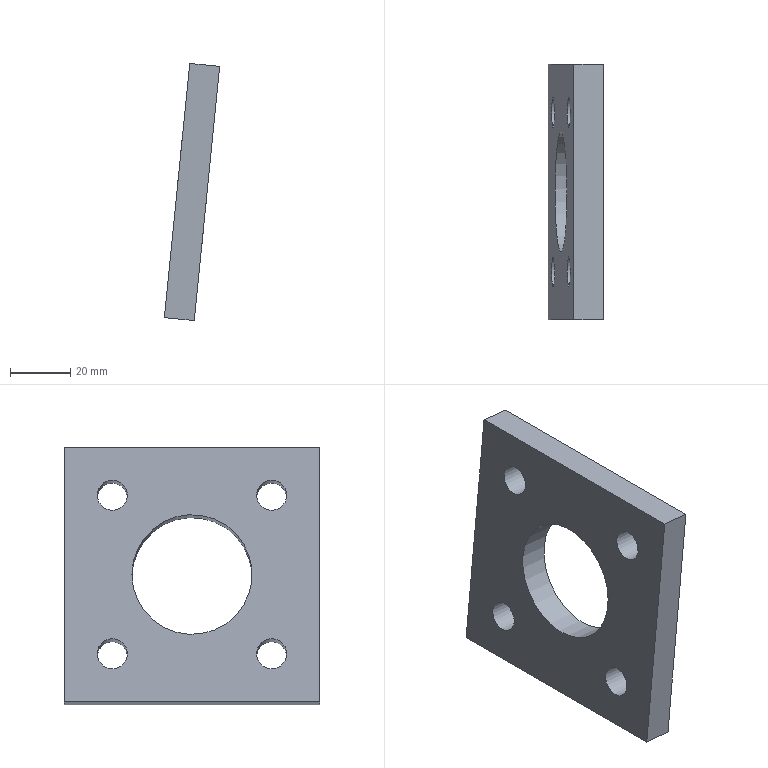Component | NX | UP_FRAME_BLOCK_2 | 1 solid | 11 faces | box 18.39 x 85 x 85.57 mm | volume 56542 mm3 | plane 6 | cylinder 5 | commonest cylinder face diameters 10 x4 40 x1
STEP:
#1=CARTESIAN_POINT('',(0.,0.,0.));
#2=DIRECTION('',(0.,0.,1.));
#3=DIRECTION('',(1.,0.,0.));
#4=AXIS2_PLACEMENT_3D('',#1,#2,#3);
#5=CARTESIAN_POINT('',(1555.629,25.,356.975));
#6=VERTEX_POINT('',#5);
#7=CARTESIAN_POINT('',(1564.071,25.,441.554));
#8=VERTEX_POINT('',#7);
#9=CARTESIAN_POINT('',(1555.629,25.,356.975));
#10=DIRECTION('',(0.09932,-0.,0.9951));
#11=VECTOR('',#10,1.);
#12=LINE('',#9,#11);
#13=CARTESIAN_POINT('',(1565.579,25.,355.981));
#14=DIRECTION('',(-0.,-1.,-0.));
#15=DIRECTION('',(-0.09932,0.,-0.9951));
#16=AXIS2_PLACEMENT_3D('',#13,#14,#15);
#17=PLANE('',#16);
#18=CARTESIAN_POINT('',(-0.,-10.));
#19=DIRECTION('',(-1.,0.));
#20=VECTOR('',#19,1.);
#21=LINE('',#18,#20);
#22=(GEOMETRIC_REPRESENTATION_CONTEXT(2)PARAMETRIC_REPRESENTATION_CONTEXT()REPRESENTATION_CONTEXT('',''));
#23=DEFINITIONAL_REPRESENTATION('',(#21),#22);
#24=PCURVE('',#17,#23);
#25=CARTESIAN_POINT('',(1562.484,94.017,425.65));
#26=DIRECTION('',(-0.9951,0.,0.09932));
#27=DIRECTION('',(0.09932,0.,0.9951));
#28=AXIS2_PLACEMENT_3D('',#25,#26,#27);
#29=PLANE('',#28);
#30=CARTESIAN_POINT('',(-69.017,-69.017));
#31=DIRECTION('',(1.,-0.));
#32=VECTOR('',#31,1.);
#33=LINE('',#30,#32);
#34=(GEOMETRIC_REPRESENTATION_CONTEXT(2)PARAMETRIC_REPRESENTATION_CONTEXT()REPRESENTATION_CONTEXT('',''));
#35=DEFINITIONAL_REPRESENTATION('',(#33),#34);
#36=PCURVE('',#29,#35);
#37=SURFACE_CURVE('',#12,(#24,#36),.PCURVE_S1.);
#38=EDGE_CURVE('',#6,#8,#37,.T.);
#39=ORIENTED_EDGE('',*,*,#38,.F.);
#40=CARTESIAN_POINT('',(1565.579,25.,355.981));
#41=VERTEX_POINT('',#40);
#42=CARTESIAN_POINT('',(1565.579,25.,355.981));
#43=DIRECTION('',(-0.9951,0.,0.09932));
#44=VECTOR('',#43,1.);
#45=LINE('',#42,#44);
#46=CARTESIAN_POINT('',(0.,0.));
#47=DIRECTION('',(0.,-1.));
#48=VECTOR('',#47,1.);
#49=LINE('',#46,#48);
#50=(GEOMETRIC_REPRESENTATION_CONTEXT(2)PARAMETRIC_REPRESENTATION_CONTEXT()REPRESENTATION_CONTEXT('',''));
#51=DEFINITIONAL_REPRESENTATION('',(#49),#50);
#52=PCURVE('',#17,#51);
#53=CARTESIAN_POINT('',(1565.579,110.,355.981));
#54=DIRECTION('',(-0.09932,0.,-0.9951));
#55=DIRECTION('',(-0.9951,0.,0.09932));
#56=AXIS2_PLACEMENT_3D('',#53,#54,#55);
#57=PLANE('',#56);
#58=CARTESIAN_POINT('',(0.,-85.));
#59=DIRECTION('',(1.,0.));
#60=VECTOR('',#59,1.);
#61=LINE('',#58,#60);
#62=(GEOMETRIC_REPRESENTATION_CONTEXT(2)PARAMETRIC_REPRESENTATION_CONTEXT()REPRESENTATION_CONTEXT('',''));
#63=DEFINITIONAL_REPRESENTATION('',(#61),#62);
#64=PCURVE('',#57,#63);
#65=SURFACE_CURVE('',#45,(#52,#64),.PCURVE_S1.);
#66=EDGE_CURVE('',#41,#6,#65,.T.);
#67=ORIENTED_EDGE('',*,*,#66,.F.);
#68=CARTESIAN_POINT('',(1574.022,25.,440.561));
#69=VERTEX_POINT('',#68);
#70=CARTESIAN_POINT('',(1565.579,25.,355.981));
#71=DIRECTION('',(0.09932,-0.,0.9951));
#72=VECTOR('',#71,1.);
#73=LINE('',#70,#72);
#74=CARTESIAN_POINT('',(0.,0.));
#75=DIRECTION('',(-1.,0.));
#76=VECTOR('',#75,1.);
#77=LINE('',#74,#76);
#78=(GEOMETRIC_REPRESENTATION_CONTEXT(2)PARAMETRIC_REPRESENTATION_CONTEXT()REPRESENTATION_CONTEXT('',''));
#79=DEFINITIONAL_REPRESENTATION('',(#77),#78);
#80=PCURVE('',#17,#79);
#81=CARTESIAN_POINT('',(1572.434,94.017,424.657));
#82=DIRECTION('',(-0.9951,0.,0.09932));
#83=DIRECTION('',(0.09932,0.,0.9951));
#84=AXIS2_PLACEMENT_3D('',#81,#82,#83);
#85=PLANE('',#84);
#86=CARTESIAN_POINT('',(-69.017,-69.017));
#87=DIRECTION('',(1.,-0.));
#88=VECTOR('',#87,1.);
#89=LINE('',#86,#88);
#90=(GEOMETRIC_REPRESENTATION_CONTEXT(2)PARAMETRIC_REPRESENTATION_CONTEXT()REPRESENTATION_CONTEXT('',''));
#91=DEFINITIONAL_REPRESENTATION('',(#89),#90);
#92=PCURVE('',#85,#91);
#93=SURFACE_CURVE('',#73,(#80,#92),.PCURVE_S1.);
#94=EDGE_CURVE('',#41,#69,#93,.T.);
#95=ORIENTED_EDGE('',*,*,#94,.T.);
#96=CARTESIAN_POINT('',(1574.022,25.,440.561));
#97=DIRECTION('',(-0.9951,0.,0.09932));
#98=VECTOR('',#97,1.);
#99=LINE('',#96,#98);
#100=CARTESIAN_POINT('',(-85.,0.));
#101=DIRECTION('',(0.,-1.));
#102=VECTOR('',#101,1.);
#103=LINE('',#100,#102);
#104=(GEOMETRIC_REPRESENTATION_CONTEXT(2)PARAMETRIC_REPRESENTATION_CONTEXT()REPRESENTATION_CONTEXT('',''));
#105=DEFINITIONAL_REPRESENTATION('',(#103),#104);
#106=PCURVE('',#17,#105);
#107=CARTESIAN_POINT('',(1574.022,25.,440.561));
#108=DIRECTION('',(0.09932,0.,0.9951));
#109=DIRECTION('',(0.9951,0.,-0.09932));
#110=AXIS2_PLACEMENT_3D('',#107,#108,#109);
#111=PLANE('',#110);
#112=CARTESIAN_POINT('',(0.,0.));
#113=DIRECTION('',(-1.,0.));
#114=VECTOR('',#113,1.);
#115=LINE('',#112,#114);
#116=(GEOMETRIC_REPRESENTATION_CONTEXT(2)PARAMETRIC_REPRESENTATION_CONTEXT()REPRESENTATION_CONTEXT('',''));
#117=DEFINITIONAL_REPRESENTATION('',(#115),#116);
#118=PCURVE('',#111,#117);
#119=SURFACE_CURVE('',#99,(#106,#118),.PCURVE_S1.);
#120=EDGE_CURVE('',#69,#8,#119,.T.);
#121=ORIENTED_EDGE('',*,*,#120,.T.);
#122=EDGE_LOOP('',(#39,#67,#95,#121));
#123=FACE_BOUND('',#122,.T.);
#124=ADVANCED_FACE('',(#123),#17,.T.);
#125=CARTESIAN_POINT('',(1564.071,110.,441.554));
#126=VERTEX_POINT('',#125);
#127=CARTESIAN_POINT('',(1564.071,25.,441.554));
#128=DIRECTION('',(0.,1.,0.));
#129=VECTOR('',#128,1.);
#130=LINE('',#127,#129);
#131=CARTESIAN_POINT('',(-10.,0.));
#132=DIRECTION('',(0.,1.));
#133=VECTOR('',#132,1.);
#134=LINE('',#131,#133);
#135=(GEOMETRIC_REPRESENTATION_CONTEXT(2)PARAMETRIC_REPRESENTATION_CONTEXT()REPRESENTATION_CONTEXT('',''));
#136=DEFINITIONAL_REPRESENTATION('',(#134),#135);
#137=PCURVE('',#111,#136);
#138=CARTESIAN_POINT('',(15.983,-69.017));
#139=DIRECTION('',(0.,1.));
#140=VECTOR('',#139,1.);
#141=LINE('',#138,#140);
#142=(GEOMETRIC_REPRESENTATION_CONTEXT(2)PARAMETRIC_REPRESENTATION_CONTEXT()REPRESENTATION_CONTEXT('',''));
#143=DEFINITIONAL_REPRESENTATION('',(#141),#142);
#144=PCURVE('',#29,#143);
#145=SURFACE_CURVE('',#130,(#137,#144),.PCURVE_S1.);
#146=EDGE_CURVE('',#8,#126,#145,.T.);
#147=ORIENTED_EDGE('',*,*,#146,.F.);
#148=ORIENTED_EDGE('',*,*,#120,.F.);
#149=CARTESIAN_POINT('',(1574.022,110.,440.561));
#150=VERTEX_POINT('',#149);
#151=CARTESIAN_POINT('',(1574.022,25.,440.561));
#152=DIRECTION('',(0.,1.,0.));
#153=VECTOR('',#152,1.);
#154=LINE('',#151,#153);
#155=CARTESIAN_POINT('',(0.,0.));
#156=DIRECTION('',(0.,1.));
#157=VECTOR('',#156,1.);
#158=LINE('',#155,#157);
#159=(GEOMETRIC_REPRESENTATION_CONTEXT(2)PARAMETRIC_REPRESENTATION_CONTEXT()REPRESENTATION_CONTEXT('',''));
#160=DEFINITIONAL_REPRESENTATION('',(#158),#159);
#161=PCURVE('',#111,#160);
#162=CARTESIAN_POINT('',(15.983,-69.017));
#163=DIRECTION('',(0.,1.));
#164=VECTOR('',#163,1.);
#165=LINE('',#162,#164);
#166=(GEOMETRIC_REPRESENTATION_CONTEXT(2)PARAMETRIC_REPRESENTATION_CONTEXT()REPRESENTATION_CONTEXT('',''));
#167=DEFINITIONAL_REPRESENTATION('',(#165),#166);
#168=PCURVE('',#85,#167);
#169=SURFACE_CURVE('',#154,(#161,#168),.PCURVE_S1.);
#170=EDGE_CURVE('',#69,#150,#169,.T.);
#171=ORIENTED_EDGE('',*,*,#170,.T.);
#172=CARTESIAN_POINT('',(1574.022,110.,440.561));
#173=DIRECTION('',(-0.9951,0.,0.09932));
#174=VECTOR('',#173,1.);
#175=LINE('',#172,#174);
#176=CARTESIAN_POINT('',(0.,85.));
#177=DIRECTION('',(-1.,0.));
#178=VECTOR('',#177,1.);
#179=LINE('',#176,#178);
#180=(GEOMETRIC_REPRESENTATION_CONTEXT(2)PARAMETRIC_REPRESENTATION_CONTEXT()REPRESENTATION_CONTEXT('',''));
#181=DEFINITIONAL_REPRESENTATION('',(#179),#180);
#182=PCURVE('',#111,#181);
#183=CARTESIAN_POINT('',(1574.022,110.,440.561));
#184=DIRECTION('',(0.,1.,0.));
#185=DIRECTION('',(0.09932,-0.,0.9951));
#186=AXIS2_PLACEMENT_3D('',#183,#184,#185);
#187=PLANE('',#186);
#188=CARTESIAN_POINT('',(0.,0.));
#189=DIRECTION('',(-0.,-1.));
#190=VECTOR('',#189,1.);
#191=LINE('',#188,#190);
#192=(GEOMETRIC_REPRESENTATION_CONTEXT(2)PARAMETRIC_REPRESENTATION_CONTEXT()REPRESENTATION_CONTEXT('',''));
#193=DEFINITIONAL_REPRESENTATION('',(#191),#192);
#194=PCURVE('',#187,#193);
#195=SURFACE_CURVE('',#175,(#182,#194),.PCURVE_S1.);
#196=EDGE_CURVE('',#150,#126,#195,.T.);
#197=ORIENTED_EDGE('',*,*,#196,.T.);
#198=EDGE_LOOP('',(#147,#148,#171,#197));
#199=FACE_BOUND('',#198,.T.);
#200=ADVANCED_FACE('',(#199),#111,.T.);
#201=CARTESIAN_POINT('',(1555.629,110.,356.975));
#202=VERTEX_POINT('',#201);
#203=CARTESIAN_POINT('',(1564.071,110.,441.554));
#204=DIRECTION('',(-0.09932,0.,-0.9951));
#205=VECTOR('',#204,1.);
#206=LINE('',#203,#205);
#207=CARTESIAN_POINT('',(0.,-10.));
#208=DIRECTION('',(-1.,0.));
#209=VECTOR('',#208,1.);
#210=LINE('',#207,#209);
#211=(GEOMETRIC_REPRESENTATION_CONTEXT(2)PARAMETRIC_REPRESENTATION_CONTEXT()REPRESENTATION_CONTEXT('',''));
#212=DEFINITIONAL_REPRESENTATION('',(#210),#211);
#213=PCURVE('',#187,#212);
#214=CARTESIAN_POINT('',(15.983,15.983));
#215=DIRECTION('',(-1.,0.));
#216=VECTOR('',#215,1.);
#217=LINE('',#214,#216);
#218=(GEOMETRIC_REPRESENTATION_CONTEXT(2)PARAMETRIC_REPRESENTATION_CONTEXT()REPRESENTATION_CONTEXT('',''));
#219=DEFINITIONAL_REPRESENTATION('',(#217),#218);
#220=PCURVE('',#29,#219);
#221=SURFACE_CURVE('',#206,(#213,#220),.PCURVE_S1.);
#222=EDGE_CURVE('',#126,#202,#221,.T.);
#223=ORIENTED_EDGE('',*,*,#222,.F.);
#224=ORIENTED_EDGE('',*,*,#196,.F.);
#225=CARTESIAN_POINT('',(1565.579,110.,355.981));
#226=VERTEX_POINT('',#225);
#227=CARTESIAN_POINT('',(1574.022,110.,440.561));
#228=DIRECTION('',(-0.09932,0.,-0.9951));
#229=VECTOR('',#228,1.);
#230=LINE('',#227,#229);
#231=CARTESIAN_POINT('',(0.,0.));
#232=DIRECTION('',(-1.,0.));
#233=VECTOR('',#232,1.);
#234=LINE('',#231,#233);
#235=(GEOMETRIC_REPRESENTATION_CONTEXT(2)PARAMETRIC_REPRESENTATION_CONTEXT()REPRESENTATION_CONTEXT('',''));
#236=DEFINITIONAL_REPRESENTATION('',(#234),#235);
#237=PCURVE('',#187,#236);
#238=CARTESIAN_POINT('',(15.983,15.983));
#239=DIRECTION('',(-1.,0.));
#240=VECTOR('',#239,1.);
#241=LINE('',#238,#240);
#242=(GEOMETRIC_REPRESENTATION_CONTEXT(2)PARAMETRIC_REPRESENTATION_CONTEXT()REPRESENTATION_CONTEXT('',''));
#243=DEFINITIONAL_REPRESENTATION('',(#241),#242);
#244=PCURVE('',#85,#243);
#245=SURFACE_CURVE('',#230,(#237,#244),.PCURVE_S1.);
#246=EDGE_CURVE('',#150,#226,#245,.T.);
#247=ORIENTED_EDGE('',*,*,#246,.T.);
#248=CARTESIAN_POINT('',(1565.579,110.,355.981));
#249=DIRECTION('',(-0.9951,0.,0.09932));
#250=VECTOR('',#249,1.);
#251=LINE('',#248,#250);
#252=CARTESIAN_POINT('',(-85.,-0.));
#253=DIRECTION('',(-0.,-1.));
#254=VECTOR('',#253,1.);
#255=LINE('',#252,#254);
#256=(GEOMETRIC_REPRESENTATION_CONTEXT(2)PARAMETRIC_REPRESENTATION_CONTEXT()REPRESENTATION_CONTEXT('',''));
#257=DEFINITIONAL_REPRESENTATION('',(#255),#256);
#258=PCURVE('',#187,#257);
#259=CARTESIAN_POINT('',(0.,0.));
#260=DIRECTION('',(1.,0.));
#261=VECTOR('',#260,1.);
#262=LINE('',#259,#261);
#263=(GEOMETRIC_REPRESENTATION_CONTEXT(2)PARAMETRIC_REPRESENTATION_CONTEXT()REPRESENTATION_CONTEXT('',''));
#264=DEFINITIONAL_REPRESENTATION('',(#262),#263);
#265=PCURVE('',#57,#264);
#266=SURFACE_CURVE('',#251,(#258,#265),.PCURVE_S1.);
#267=EDGE_CURVE('',#226,#202,#266,.T.);
#268=ORIENTED_EDGE('',*,*,#267,.T.);
#269=EDGE_LOOP('',(#223,#224,#247,#268));
#270=FACE_BOUND('',#269,.T.);
#271=ADVANCED_FACE('',(#270),#187,.T.);
#272=CARTESIAN_POINT('',(1572.434,45.983,424.657));
#273=VERTEX_POINT('',#272);
#274=CARTESIAN_POINT('',(1572.434,40.983,424.657));
#275=DIRECTION('',(0.9951,0.,-0.09932));
#276=DIRECTION('',(0.,1.,0.));
#277=AXIS2_PLACEMENT_3D('',#274,#275,#276);
#278=CIRCLE('',#277,5.);
#279=CARTESIAN_POINT('',(1572.434,40.983,424.657));
#280=DIRECTION('',(-0.9951,0.,0.09932));
#281=DIRECTION('',(0.09932,0.,0.9951));
#282=AXIS2_PLACEMENT_3D('',#279,#280,#281);
#283=CYLINDRICAL_SURFACE('',#282,5.);
#284=CARTESIAN_POINT('',(7.854,0.));
#285=DIRECTION('',(-1.,0.));
#286=VECTOR('',#285,1.);
#287=LINE('',#284,#286);
#288=(GEOMETRIC_REPRESENTATION_CONTEXT(2)PARAMETRIC_REPRESENTATION_CONTEXT()REPRESENTATION_CONTEXT('',''));
#289=DEFINITIONAL_REPRESENTATION('',(#287),#288);
#290=PCURVE('',#283,#289);
#291=CARTESIAN_POINT('',(0.,-48.033));
#292=CARTESIAN_POINT('',(8.66,-48.033));
#293=CARTESIAN_POINT('',(4.33,-55.533));
#294=CARTESIAN_POINT('',(0.,-63.033));
#295=CARTESIAN_POINT('',(-4.33,-55.533));
#296=CARTESIAN_POINT('',(-8.66,-48.033));
#297=CARTESIAN_POINT('',(0.,-48.033));
#298=(BOUNDED_CURVE()B_SPLINE_CURVE(2,(#291,#292,#293,#294,#295,#296,#297),.UNSPECIFIED.,.T.,.F.)B_SPLINE_CURVE_WITH_KNOTS((1,2,2,2,2,1),(-2.094,0.,2.094,4.189,6.283,8.378),.UNSPECIFIED.)CURVE()GEOMETRIC_REPRESENTATION_ITEM()RATIONAL_B_SPLINE_CURVE((1.,0.5,1.,0.5,1.,0.5,1.))REPRESENTATION_ITEM(''));
#299=(GEOMETRIC_REPRESENTATION_CONTEXT(2)PARAMETRIC_REPRESENTATION_CONTEXT()REPRESENTATION_CONTEXT('',''));
#300=DEFINITIONAL_REPRESENTATION('',(#298),#299);
#301=PCURVE('',#85,#300);
#302=SURFACE_CURVE('',#278,(#290,#301),.PCURVE_S1.);
#303=EDGE_CURVE('',#273,#273,#302,.T.);
#304=ORIENTED_EDGE('',*,*,#303,.F.);
#305=CARTESIAN_POINT('',(1562.484,45.983,425.65));
#306=VERTEX_POINT('',#305);
#307=CARTESIAN_POINT('',(1572.434,45.983,424.657));
#308=CARTESIAN_POINT('',(1562.484,45.983,425.65));
#309=B_SPLINE_CURVE_WITH_KNOTS('',1,(#307,#308),.UNSPECIFIED.,.F.,.F.,(2,2),(0.,10.),.PIECEWISE_BEZIER_KNOTS.);
#310=CARTESIAN_POINT('',(7.854,0.));
#311=DIRECTION('',(0.,1.));
#312=VECTOR('',#311,1.);
#313=LINE('',#310,#312);
#314=(GEOMETRIC_REPRESENTATION_CONTEXT(2)PARAMETRIC_REPRESENTATION_CONTEXT()REPRESENTATION_CONTEXT('',''));
#315=DEFINITIONAL_REPRESENTATION('',(#313),#314);
#316=PCURVE('',#283,#315);
#317=CARTESIAN_POINT('',(1.571,0.));
#318=DIRECTION('',(0.,1.));
#319=VECTOR('',#318,1.);
#320=LINE('',#317,#319);
#321=(GEOMETRIC_REPRESENTATION_CONTEXT(2)PARAMETRIC_REPRESENTATION_CONTEXT()REPRESENTATION_CONTEXT('',''));
#322=DEFINITIONAL_REPRESENTATION('',(#320),#321);
#323=PCURVE('',#283,#322);
#324=SEAM_CURVE('',#309,(#316,#323),.PCURVE_S1.);
#325=EDGE_CURVE('',#273,#306,#324,.T.);
#326=ORIENTED_EDGE('',*,*,#325,.T.);
#327=CARTESIAN_POINT('',(1562.484,40.983,425.65));
#328=DIRECTION('',(0.9951,0.,-0.09932));
#329=DIRECTION('',(0.,1.,0.));
#330=AXIS2_PLACEMENT_3D('',#327,#328,#329);
#331=CIRCLE('',#330,5.);
#332=CARTESIAN_POINT('',(7.854,10.));
#333=DIRECTION('',(-1.,0.));
#334=VECTOR('',#333,1.);
#335=LINE('',#332,#334);
#336=(GEOMETRIC_REPRESENTATION_CONTEXT(2)PARAMETRIC_REPRESENTATION_CONTEXT()REPRESENTATION_CONTEXT('',''));
#337=DEFINITIONAL_REPRESENTATION('',(#335),#336);
#338=PCURVE('',#283,#337);
#339=CARTESIAN_POINT('',(0.,-48.033));
#340=CARTESIAN_POINT('',(8.66,-48.033));
#341=CARTESIAN_POINT('',(4.33,-55.533));
#342=CARTESIAN_POINT('',(0.,-63.033));
#343=CARTESIAN_POINT('',(-4.33,-55.533));
#344=CARTESIAN_POINT('',(-8.66,-48.033));
#345=CARTESIAN_POINT('',(0.,-48.033));
#346=(BOUNDED_CURVE()B_SPLINE_CURVE(2,(#339,#340,#341,#342,#343,#344,#345),.UNSPECIFIED.,.T.,.F.)B_SPLINE_CURVE_WITH_KNOTS((1,2,2,2,2,1),(-2.094,0.,2.094,4.189,6.283,8.378),.UNSPECIFIED.)CURVE()GEOMETRIC_REPRESENTATION_ITEM()RATIONAL_B_SPLINE_CURVE((1.,0.5,1.,0.5,1.,0.5,1.))REPRESENTATION_ITEM(''));
#347=(GEOMETRIC_REPRESENTATION_CONTEXT(2)PARAMETRIC_REPRESENTATION_CONTEXT()REPRESENTATION_CONTEXT('',''));
#348=DEFINITIONAL_REPRESENTATION('',(#346),#347);
#349=PCURVE('',#29,#348);
#350=SURFACE_CURVE('',#331,(#338,#349),.PCURVE_S1.);
#351=EDGE_CURVE('',#306,#306,#350,.T.);
#352=ORIENTED_EDGE('',*,*,#351,.T.);
#353=ORIENTED_EDGE('',*,*,#325,.F.);
#354=EDGE_LOOP('',(#304,#326,#352,#353));
#355=FACE_BOUND('',#354,.F.);
#356=ADVANCED_FACE('',(#355),#283,.F.);
#357=CARTESIAN_POINT('',(1567.167,89.017,371.886));
#358=VERTEX_POINT('',#357);
#359=CARTESIAN_POINT('',(1567.167,94.017,371.886));
#360=DIRECTION('',(0.9951,0.,-0.09932));
#361=DIRECTION('',(0.,-1.,0.));
#362=AXIS2_PLACEMENT_3D('',#359,#360,#361);
#363=CIRCLE('',#362,5.);
#364=CARTESIAN_POINT('',(1567.167,94.017,371.886));
#365=DIRECTION('',(-0.9951,0.,0.09932));
#366=DIRECTION('',(0.09932,0.,0.9951));
#367=AXIS2_PLACEMENT_3D('',#364,#365,#366);
#368=CYLINDRICAL_SURFACE('',#367,5.);
#369=CARTESIAN_POINT('',(10.996,0.));
#370=DIRECTION('',(-1.,0.));
#371=VECTOR('',#370,1.);
#372=LINE('',#369,#371);
#373=(GEOMETRIC_REPRESENTATION_CONTEXT(2)PARAMETRIC_REPRESENTATION_CONTEXT()REPRESENTATION_CONTEXT('',''));
#374=DEFINITIONAL_REPRESENTATION('',(#372),#373);
#375=PCURVE('',#368,#374);
#376=CARTESIAN_POINT('',(-53.033,-5.));
#377=CARTESIAN_POINT('',(-61.693,-5.));
#378=CARTESIAN_POINT('',(-57.363,2.5));
#379=CARTESIAN_POINT('',(-53.033,10.));
#380=CARTESIAN_POINT('',(-48.703,2.5));
#381=CARTESIAN_POINT('',(-44.373,-5.));
#382=CARTESIAN_POINT('',(-53.033,-5.));
#383=(BOUNDED_CURVE()B_SPLINE_CURVE(2,(#376,#377,#378,#379,#380,#381,#382),.UNSPECIFIED.,.T.,.F.)B_SPLINE_CURVE_WITH_KNOTS((1,2,2,2,2,1),(-2.094,0.,2.094,4.189,6.283,8.378),.UNSPECIFIED.)CURVE()GEOMETRIC_REPRESENTATION_ITEM()RATIONAL_B_SPLINE_CURVE((1.,0.5,1.,0.5,1.,0.5,1.))REPRESENTATION_ITEM(''));
#384=(GEOMETRIC_REPRESENTATION_CONTEXT(2)PARAMETRIC_REPRESENTATION_CONTEXT()REPRESENTATION_CONTEXT('',''));
#385=DEFINITIONAL_REPRESENTATION('',(#383),#384);
#386=PCURVE('',#85,#385);
#387=SURFACE_CURVE('',#363,(#375,#386),.PCURVE_S1.);
#388=EDGE_CURVE('',#358,#358,#387,.T.);
#389=ORIENTED_EDGE('',*,*,#388,.F.);
#390=CARTESIAN_POINT('',(1557.216,89.017,372.879));
#391=VERTEX_POINT('',#390);
#392=CARTESIAN_POINT('',(1567.167,89.017,371.886));
#393=CARTESIAN_POINT('',(1557.216,89.017,372.879));
#394=B_SPLINE_CURVE_WITH_KNOTS('',1,(#392,#393),.UNSPECIFIED.,.F.,.F.,(2,2),(0.,10.),.PIECEWISE_BEZIER_KNOTS.);
#395=CARTESIAN_POINT('',(10.996,0.));
#396=DIRECTION('',(0.,1.));
#397=VECTOR('',#396,1.);
#398=LINE('',#395,#397);
#399=(GEOMETRIC_REPRESENTATION_CONTEXT(2)PARAMETRIC_REPRESENTATION_CONTEXT()REPRESENTATION_CONTEXT('',''));
#400=DEFINITIONAL_REPRESENTATION('',(#398),#399);
#401=PCURVE('',#368,#400);
#402=CARTESIAN_POINT('',(4.712,0.));
#403=DIRECTION('',(0.,1.));
#404=VECTOR('',#403,1.);
#405=LINE('',#402,#404);
#406=(GEOMETRIC_REPRESENTATION_CONTEXT(2)PARAMETRIC_REPRESENTATION_CONTEXT()REPRESENTATION_CONTEXT('',''));
#407=DEFINITIONAL_REPRESENTATION('',(#405),#406);
#408=PCURVE('',#368,#407);
#409=SEAM_CURVE('',#394,(#401,#408),.PCURVE_S1.);
#410=EDGE_CURVE('',#358,#391,#409,.T.);
#411=ORIENTED_EDGE('',*,*,#410,.T.);
#412=CARTESIAN_POINT('',(1557.216,94.017,372.879));
#413=DIRECTION('',(0.9951,0.,-0.09932));
#414=DIRECTION('',(0.,-1.,0.));
#415=AXIS2_PLACEMENT_3D('',#412,#413,#414);
#416=CIRCLE('',#415,5.);
#417=CARTESIAN_POINT('',(10.996,10.));
#418=DIRECTION('',(-1.,0.));
#419=VECTOR('',#418,1.);
#420=LINE('',#417,#419);
#421=(GEOMETRIC_REPRESENTATION_CONTEXT(2)PARAMETRIC_REPRESENTATION_CONTEXT()REPRESENTATION_CONTEXT('',''));
#422=DEFINITIONAL_REPRESENTATION('',(#420),#421);
#423=PCURVE('',#368,#422);
#424=CARTESIAN_POINT('',(-53.033,-5.));
#425=CARTESIAN_POINT('',(-61.693,-5.));
#426=CARTESIAN_POINT('',(-57.363,2.5));
#427=CARTESIAN_POINT('',(-53.033,10.));
#428=CARTESIAN_POINT('',(-48.703,2.5));
#429=CARTESIAN_POINT('',(-44.373,-5.));
#430=CARTESIAN_POINT('',(-53.033,-5.));
#431=(BOUNDED_CURVE()B_SPLINE_CURVE(2,(#424,#425,#426,#427,#428,#429,#430),.UNSPECIFIED.,.T.,.F.)B_SPLINE_CURVE_WITH_KNOTS((1,2,2,2,2,1),(-2.094,0.,2.094,4.189,6.283,8.378),.UNSPECIFIED.)CURVE()GEOMETRIC_REPRESENTATION_ITEM()RATIONAL_B_SPLINE_CURVE((1.,0.5,1.,0.5,1.,0.5,1.))REPRESENTATION_ITEM(''));
#432=(GEOMETRIC_REPRESENTATION_CONTEXT(2)PARAMETRIC_REPRESENTATION_CONTEXT()REPRESENTATION_CONTEXT('',''));
#433=DEFINITIONAL_REPRESENTATION('',(#431),#432);
#434=PCURVE('',#29,#433);
#435=SURFACE_CURVE('',#416,(#423,#434),.PCURVE_S1.);
#436=EDGE_CURVE('',#391,#391,#435,.T.);
#437=ORIENTED_EDGE('',*,*,#436,.T.);
#438=ORIENTED_EDGE('',*,*,#410,.F.);
#439=EDGE_LOOP('',(#389,#411,#437,#438));
#440=FACE_BOUND('',#439,.F.);
#441=ADVANCED_FACE('',(#440),#368,.F.);
#442=CARTESIAN_POINT('',(1569.8,87.5,398.271));
#443=VERTEX_POINT('',#442);
#444=CARTESIAN_POINT('',(1569.8,67.5,398.271));
#445=DIRECTION('',(0.9951,0.,-0.09932));
#446=DIRECTION('',(0.,1.,0.));
#447=AXIS2_PLACEMENT_3D('',#444,#445,#446);
#448=CIRCLE('',#447,20.);
#449=CARTESIAN_POINT('',(1569.8,67.5,398.271));
#450=DIRECTION('',(-0.9951,0.,0.09932));
#451=DIRECTION('',(0.09932,0.,0.9951));
#452=AXIS2_PLACEMENT_3D('',#449,#450,#451);
#453=CYLINDRICAL_SURFACE('',#452,20.);
#454=CARTESIAN_POINT('',(7.854,0.));
#455=DIRECTION('',(-1.,0.));
#456=VECTOR('',#455,1.);
#457=LINE('',#454,#456);
#458=(GEOMETRIC_REPRESENTATION_CONTEXT(2)PARAMETRIC_REPRESENTATION_CONTEXT()REPRESENTATION_CONTEXT('',''));
#459=DEFINITIONAL_REPRESENTATION('',(#457),#458);
#460=PCURVE('',#453,#459);
#461=CARTESIAN_POINT('',(-26.517,-6.517));
#462=CARTESIAN_POINT('',(8.125,-6.517));
#463=CARTESIAN_POINT('',(-9.196,-36.517));
#464=CARTESIAN_POINT('',(-26.517,-66.517));
#465=CARTESIAN_POINT('',(-43.837,-36.517));
#466=CARTESIAN_POINT('',(-61.158,-6.517));
#467=CARTESIAN_POINT('',(-26.517,-6.517));
#468=(BOUNDED_CURVE()B_SPLINE_CURVE(2,(#461,#462,#463,#464,#465,#466,#467),.UNSPECIFIED.,.T.,.F.)B_SPLINE_CURVE_WITH_KNOTS((1,2,2,2,2,1),(-2.094,0.,2.094,4.189,6.283,8.378),.UNSPECIFIED.)CURVE()GEOMETRIC_REPRESENTATION_ITEM()RATIONAL_B_SPLINE_CURVE((1.,0.5,1.,0.5,1.,0.5,1.))REPRESENTATION_ITEM(''));
#469=(GEOMETRIC_REPRESENTATION_CONTEXT(2)PARAMETRIC_REPRESENTATION_CONTEXT()REPRESENTATION_CONTEXT('',''));
#470=DEFINITIONAL_REPRESENTATION('',(#468),#469);
#471=PCURVE('',#85,#470);
#472=SURFACE_CURVE('',#448,(#460,#471),.PCURVE_S1.);
#473=EDGE_CURVE('',#443,#443,#472,.T.);
#474=ORIENTED_EDGE('',*,*,#473,.F.);
#475=CARTESIAN_POINT('',(1559.85,87.5,399.265));
#476=VERTEX_POINT('',#475);
#477=CARTESIAN_POINT('',(1569.8,87.5,398.271));
#478=CARTESIAN_POINT('',(1559.85,87.5,399.265));
#479=B_SPLINE_CURVE_WITH_KNOTS('',1,(#477,#478),.UNSPECIFIED.,.F.,.F.,(2,2),(0.,10.),.PIECEWISE_BEZIER_KNOTS.);
#480=CARTESIAN_POINT('',(7.854,0.));
#481=DIRECTION('',(0.,1.));
#482=VECTOR('',#481,1.);
#483=LINE('',#480,#482);
#484=(GEOMETRIC_REPRESENTATION_CONTEXT(2)PARAMETRIC_REPRESENTATION_CONTEXT()REPRESENTATION_CONTEXT('',''));
#485=DEFINITIONAL_REPRESENTATION('',(#483),#484);
#486=PCURVE('',#453,#485);
#487=CARTESIAN_POINT('',(1.571,0.));
#488=DIRECTION('',(0.,1.));
#489=VECTOR('',#488,1.);
#490=LINE('',#487,#489);
#491=(GEOMETRIC_REPRESENTATION_CONTEXT(2)PARAMETRIC_REPRESENTATION_CONTEXT()REPRESENTATION_CONTEXT('',''));
#492=DEFINITIONAL_REPRESENTATION('',(#490),#491);
#493=PCURVE('',#453,#492);
#494=SEAM_CURVE('',#479,(#486,#493),.PCURVE_S1.);
#495=EDGE_CURVE('',#443,#476,#494,.T.);
#496=ORIENTED_EDGE('',*,*,#495,.T.);
#497=CARTESIAN_POINT('',(1559.85,67.5,399.265));
#498=DIRECTION('',(0.9951,0.,-0.09932));
#499=DIRECTION('',(0.,1.,0.));
#500=AXIS2_PLACEMENT_3D('',#497,#498,#499);
#501=CIRCLE('',#500,20.);
#502=CARTESIAN_POINT('',(7.854,10.));
#503=DIRECTION('',(-1.,0.));
#504=VECTOR('',#503,1.);
#505=LINE('',#502,#504);
#506=(GEOMETRIC_REPRESENTATION_CONTEXT(2)PARAMETRIC_REPRESENTATION_CONTEXT()REPRESENTATION_CONTEXT('',''));
#507=DEFINITIONAL_REPRESENTATION('',(#505),#506);
#508=PCURVE('',#453,#507);
#509=CARTESIAN_POINT('',(-26.517,-6.517));
#510=CARTESIAN_POINT('',(8.125,-6.517));
#511=CARTESIAN_POINT('',(-9.196,-36.517));
#512=CARTESIAN_POINT('',(-26.517,-66.517));
#513=CARTESIAN_POINT('',(-43.837,-36.517));
#514=CARTESIAN_POINT('',(-61.158,-6.517));
#515=CARTESIAN_POINT('',(-26.517,-6.517));
#516=(BOUNDED_CURVE()B_SPLINE_CURVE(2,(#509,#510,#511,#512,#513,#514,#515),.UNSPECIFIED.,.T.,.F.)B_SPLINE_CURVE_WITH_KNOTS((1,2,2,2,2,1),(-2.094,0.,2.094,4.189,6.283,8.378),.UNSPECIFIED.)CURVE()GEOMETRIC_REPRESENTATION_ITEM()RATIONAL_B_SPLINE_CURVE((1.,0.5,1.,0.5,1.,0.5,1.))REPRESENTATION_ITEM(''));
#517=(GEOMETRIC_REPRESENTATION_CONTEXT(2)PARAMETRIC_REPRESENTATION_CONTEXT()REPRESENTATION_CONTEXT('',''));
#518=DEFINITIONAL_REPRESENTATION('',(#516),#517);
#519=PCURVE('',#29,#518);
#520=SURFACE_CURVE('',#501,(#508,#519),.PCURVE_S1.);
#521=EDGE_CURVE('',#476,#476,#520,.T.);
#522=ORIENTED_EDGE('',*,*,#521,.T.);
#523=ORIENTED_EDGE('',*,*,#495,.F.);
#524=EDGE_LOOP('',(#474,#496,#522,#523));
#525=FACE_BOUND('',#524,.F.);
#526=ADVANCED_FACE('',(#525),#453,.F.);
#527=CARTESIAN_POINT('',(1572.434,89.017,424.657));
#528=VERTEX_POINT('',#527);
#529=CARTESIAN_POINT('',(1572.434,94.017,424.657));
#530=DIRECTION('',(-0.9951,0.,0.09932));
#531=DIRECTION('',(0.,-1.,0.));
#532=AXIS2_PLACEMENT_3D('',#529,#530,#531);
#533=CIRCLE('',#532,5.);
#534=CARTESIAN_POINT('',(1572.434,94.017,424.657));
#535=DIRECTION('',(-0.9951,0.,0.09932));
#536=DIRECTION('',(0.09932,0.,0.9951));
#537=AXIS2_PLACEMENT_3D('',#534,#535,#536);
#538=CYLINDRICAL_SURFACE('',#537,5.);
#539=CARTESIAN_POINT('',(4.712,0.));
#540=DIRECTION('',(1.,0.));
#541=VECTOR('',#540,1.);
#542=LINE('',#539,#541);
#543=(GEOMETRIC_REPRESENTATION_CONTEXT(2)PARAMETRIC_REPRESENTATION_CONTEXT()REPRESENTATION_CONTEXT('',''));
#544=DEFINITIONAL_REPRESENTATION('',(#542),#543);
#545=PCURVE('',#538,#544);
#546=CARTESIAN_POINT('',(0.,0.));
#547=DIRECTION('',(0.,-1.));
#548=AXIS2_PLACEMENT_2D('',#546,#547);
#549=CIRCLE('',#548,5.);
#550=(GEOMETRIC_REPRESENTATION_CONTEXT(2)PARAMETRIC_REPRESENTATION_CONTEXT()REPRESENTATION_CONTEXT('',''));
#551=DEFINITIONAL_REPRESENTATION('',(#549),#550);
#552=PCURVE('',#85,#551);
#553=SURFACE_CURVE('',#533,(#545,#552),.PCURVE_S1.);
#554=EDGE_CURVE('',#528,#528,#553,.T.);
#555=ORIENTED_EDGE('',*,*,#554,.T.);
#556=CARTESIAN_POINT('',(1562.484,89.017,425.65));
#557=VERTEX_POINT('',#556);
#558=CARTESIAN_POINT('',(1572.434,89.017,424.657));
#559=CARTESIAN_POINT('',(1562.484,89.017,425.65));
#560=B_SPLINE_CURVE_WITH_KNOTS('',1,(#558,#559),.UNSPECIFIED.,.F.,.F.,(2,2),(0.,10.),.PIECEWISE_BEZIER_KNOTS.);
#561=CARTESIAN_POINT('',(10.996,0.));
#562=DIRECTION('',(0.,1.));
#563=VECTOR('',#562,1.);
#564=LINE('',#561,#563);
#565=(GEOMETRIC_REPRESENTATION_CONTEXT(2)PARAMETRIC_REPRESENTATION_CONTEXT()REPRESENTATION_CONTEXT('',''));
#566=DEFINITIONAL_REPRESENTATION('',(#564),#565);
#567=PCURVE('',#538,#566);
#568=CARTESIAN_POINT('',(4.712,0.));
#569=DIRECTION('',(0.,1.));
#570=VECTOR('',#569,1.);
#571=LINE('',#568,#570);
#572=(GEOMETRIC_REPRESENTATION_CONTEXT(2)PARAMETRIC_REPRESENTATION_CONTEXT()REPRESENTATION_CONTEXT('',''));
#573=DEFINITIONAL_REPRESENTATION('',(#571),#572);
#574=PCURVE('',#538,#573);
#575=SEAM_CURVE('',#560,(#567,#574),.PCURVE_S1.);
#576=EDGE_CURVE('',#528,#557,#575,.T.);
#577=ORIENTED_EDGE('',*,*,#576,.T.);
#578=CARTESIAN_POINT('',(1562.484,94.017,425.65));
#579=DIRECTION('',(-0.9951,0.,0.09932));
#580=DIRECTION('',(0.,-1.,0.));
#581=AXIS2_PLACEMENT_3D('',#578,#579,#580);
#582=CIRCLE('',#581,5.);
#583=CARTESIAN_POINT('',(4.712,10.));
#584=DIRECTION('',(1.,0.));
#585=VECTOR('',#584,1.);
#586=LINE('',#583,#585);
#587=(GEOMETRIC_REPRESENTATION_CONTEXT(2)PARAMETRIC_REPRESENTATION_CONTEXT()REPRESENTATION_CONTEXT('',''));
#588=DEFINITIONAL_REPRESENTATION('',(#586),#587);
#589=PCURVE('',#538,#588);
#590=CARTESIAN_POINT('',(0.,0.));
#591=DIRECTION('',(0.,-1.));
#592=AXIS2_PLACEMENT_2D('',#590,#591);
#593=CIRCLE('',#592,5.);
#594=(GEOMETRIC_REPRESENTATION_CONTEXT(2)PARAMETRIC_REPRESENTATION_CONTEXT()REPRESENTATION_CONTEXT('',''));
#595=DEFINITIONAL_REPRESENTATION('',(#593),#594);
#596=PCURVE('',#29,#595);
#597=SURFACE_CURVE('',#582,(#589,#596),.PCURVE_S1.);
#598=EDGE_CURVE('',#557,#557,#597,.T.);
#599=ORIENTED_EDGE('',*,*,#598,.F.);
#600=ORIENTED_EDGE('',*,*,#576,.F.);
#601=EDGE_LOOP('',(#555,#577,#599,#600));
#602=FACE_BOUND('',#601,.F.);
#603=ADVANCED_FACE('',(#602),#538,.F.);
#604=CARTESIAN_POINT('',(1555.629,110.,356.975));
#605=DIRECTION('',(0.,-1.,0.));
#606=VECTOR('',#605,1.);
#607=LINE('',#604,#606);
#608=CARTESIAN_POINT('',(10.,0.));
#609=DIRECTION('',(0.,-1.));
#610=VECTOR('',#609,1.);
#611=LINE('',#608,#610);
#612=(GEOMETRIC_REPRESENTATION_CONTEXT(2)PARAMETRIC_REPRESENTATION_CONTEXT()REPRESENTATION_CONTEXT('',''));
#613=DEFINITIONAL_REPRESENTATION('',(#611),#612);
#614=PCURVE('',#57,#613);
#615=CARTESIAN_POINT('',(-69.017,15.983));
#616=DIRECTION('',(0.,-1.));
#617=VECTOR('',#616,1.);
#618=LINE('',#615,#617);
#619=(GEOMETRIC_REPRESENTATION_CONTEXT(2)PARAMETRIC_REPRESENTATION_CONTEXT()REPRESENTATION_CONTEXT('',''));
#620=DEFINITIONAL_REPRESENTATION('',(#618),#619);
#621=PCURVE('',#29,#620);
#622=SURFACE_CURVE('',#607,(#614,#621),.PCURVE_S1.);
#623=EDGE_CURVE('',#202,#6,#622,.T.);
#624=ORIENTED_EDGE('',*,*,#623,.F.);
#625=ORIENTED_EDGE('',*,*,#267,.F.);
#626=CARTESIAN_POINT('',(1565.579,110.,355.981));
#627=DIRECTION('',(0.,-1.,0.));
#628=VECTOR('',#627,1.);
#629=LINE('',#626,#628);
#630=CARTESIAN_POINT('',(0.,0.));
#631=DIRECTION('',(0.,-1.));
#632=VECTOR('',#631,1.);
#633=LINE('',#630,#632);
#634=(GEOMETRIC_REPRESENTATION_CONTEXT(2)PARAMETRIC_REPRESENTATION_CONTEXT()REPRESENTATION_CONTEXT('',''));
#635=DEFINITIONAL_REPRESENTATION('',(#633),#634);
#636=PCURVE('',#57,#635);
#637=CARTESIAN_POINT('',(-69.017,15.983));
#638=DIRECTION('',(0.,-1.));
#639=VECTOR('',#638,1.);
#640=LINE('',#637,#639);
#641=(GEOMETRIC_REPRESENTATION_CONTEXT(2)PARAMETRIC_REPRESENTATION_CONTEXT()REPRESENTATION_CONTEXT('',''));
#642=DEFINITIONAL_REPRESENTATION('',(#640),#641);
#643=PCURVE('',#85,#642);
#644=SURFACE_CURVE('',#629,(#636,#643),.PCURVE_S1.);
#645=EDGE_CURVE('',#226,#41,#644,.T.);
#646=ORIENTED_EDGE('',*,*,#645,.T.);
#647=ORIENTED_EDGE('',*,*,#66,.T.);
#648=EDGE_LOOP('',(#624,#625,#646,#647));
#649=FACE_BOUND('',#648,.T.);
#650=ADVANCED_FACE('',(#649),#57,.T.);
#651=CARTESIAN_POINT('',(1567.167,45.983,371.886));
#652=VERTEX_POINT('',#651);
#653=CARTESIAN_POINT('',(1567.167,40.983,371.886));
#654=DIRECTION('',(-0.9951,0.,0.09932));
#655=DIRECTION('',(0.,1.,0.));
#656=AXIS2_PLACEMENT_3D('',#653,#654,#655);
#657=CIRCLE('',#656,5.);
#658=CARTESIAN_POINT('',(1567.167,40.983,371.886));
#659=DIRECTION('',(-0.9951,0.,0.09932));
#660=DIRECTION('',(0.09932,0.,0.9951));
#661=AXIS2_PLACEMENT_3D('',#658,#659,#660);
#662=CYLINDRICAL_SURFACE('',#661,5.);
#663=CARTESIAN_POINT('',(1.571,0.));
#664=DIRECTION('',(1.,0.));
#665=VECTOR('',#664,1.);
#666=LINE('',#663,#665);
#667=(GEOMETRIC_REPRESENTATION_CONTEXT(2)PARAMETRIC_REPRESENTATION_CONTEXT()REPRESENTATION_CONTEXT('',''));
#668=DEFINITIONAL_REPRESENTATION('',(#666),#667);
#669=PCURVE('',#662,#668);
#670=CARTESIAN_POINT('',(-53.033,-53.033));
#671=DIRECTION('',(0.,1.));
#672=AXIS2_PLACEMENT_2D('',#670,#671);
#673=CIRCLE('',#672,5.);
#674=(GEOMETRIC_REPRESENTATION_CONTEXT(2)PARAMETRIC_REPRESENTATION_CONTEXT()REPRESENTATION_CONTEXT('',''));
#675=DEFINITIONAL_REPRESENTATION('',(#673),#674);
#676=PCURVE('',#85,#675);
#677=SURFACE_CURVE('',#657,(#669,#676),.PCURVE_S1.);
#678=EDGE_CURVE('',#652,#652,#677,.T.);
#679=ORIENTED_EDGE('',*,*,#678,.T.);
#680=CARTESIAN_POINT('',(1557.216,45.983,372.879));
#681=VERTEX_POINT('',#680);
#682=CARTESIAN_POINT('',(1567.167,45.983,371.886));
#683=CARTESIAN_POINT('',(1557.216,45.983,372.879));
#684=B_SPLINE_CURVE_WITH_KNOTS('',1,(#682,#683),.UNSPECIFIED.,.F.,.F.,(2,2),(0.,10.),.PIECEWISE_BEZIER_KNOTS.);
#685=CARTESIAN_POINT('',(7.854,0.));
#686=DIRECTION('',(0.,1.));
#687=VECTOR('',#686,1.);
#688=LINE('',#685,#687);
#689=(GEOMETRIC_REPRESENTATION_CONTEXT(2)PARAMETRIC_REPRESENTATION_CONTEXT()REPRESENTATION_CONTEXT('',''));
#690=DEFINITIONAL_REPRESENTATION('',(#688),#689);
#691=PCURVE('',#662,#690);
#692=CARTESIAN_POINT('',(1.571,0.));
#693=DIRECTION('',(0.,1.));
#694=VECTOR('',#693,1.);
#695=LINE('',#692,#694);
#696=(GEOMETRIC_REPRESENTATION_CONTEXT(2)PARAMETRIC_REPRESENTATION_CONTEXT()REPRESENTATION_CONTEXT('',''));
#697=DEFINITIONAL_REPRESENTATION('',(#695),#696);
#698=PCURVE('',#662,#697);
#699=SEAM_CURVE('',#684,(#691,#698),.PCURVE_S1.);
#700=EDGE_CURVE('',#652,#681,#699,.T.);
#701=ORIENTED_EDGE('',*,*,#700,.T.);
#702=CARTESIAN_POINT('',(1557.216,40.983,372.879));
#703=DIRECTION('',(-0.9951,0.,0.09932));
#704=DIRECTION('',(0.,1.,0.));
#705=AXIS2_PLACEMENT_3D('',#702,#703,#704);
#706=CIRCLE('',#705,5.);
#707=CARTESIAN_POINT('',(1.571,10.));
#708=DIRECTION('',(1.,0.));
#709=VECTOR('',#708,1.);
#710=LINE('',#707,#709);
#711=(GEOMETRIC_REPRESENTATION_CONTEXT(2)PARAMETRIC_REPRESENTATION_CONTEXT()REPRESENTATION_CONTEXT('',''));
#712=DEFINITIONAL_REPRESENTATION('',(#710),#711);
#713=PCURVE('',#662,#712);
#714=CARTESIAN_POINT('',(-53.033,-53.033));
#715=DIRECTION('',(0.,1.));
#716=AXIS2_PLACEMENT_2D('',#714,#715);
#717=CIRCLE('',#716,5.);
#718=(GEOMETRIC_REPRESENTATION_CONTEXT(2)PARAMETRIC_REPRESENTATION_CONTEXT()REPRESENTATION_CONTEXT('',''));
#719=DEFINITIONAL_REPRESENTATION('',(#717),#718);
#720=PCURVE('',#29,#719);
#721=SURFACE_CURVE('',#706,(#713,#720),.PCURVE_S1.);
#722=EDGE_CURVE('',#681,#681,#721,.T.);
#723=ORIENTED_EDGE('',*,*,#722,.F.);
#724=ORIENTED_EDGE('',*,*,#700,.F.);
#725=EDGE_LOOP('',(#679,#701,#723,#724));
#726=FACE_BOUND('',#725,.F.);
#727=ADVANCED_FACE('',(#726),#662,.F.);
#728=ORIENTED_EDGE('',*,*,#94,.F.);
#729=ORIENTED_EDGE('',*,*,#645,.F.);
#730=ORIENTED_EDGE('',*,*,#246,.F.);
#731=ORIENTED_EDGE('',*,*,#170,.F.);
#732=EDGE_LOOP('',(#728,#729,#730,#731));
#733=FACE_BOUND('',#732,.T.);
#734=ORIENTED_EDGE('',*,*,#554,.T.);
#735=EDGE_LOOP('',(#734));
#736=FACE_BOUND('',#735,.T.);
#737=ORIENTED_EDGE('',*,*,#473,.F.);
#738=EDGE_LOOP('',(#737));
#739=FACE_BOUND('',#738,.T.);
#740=ORIENTED_EDGE('',*,*,#388,.F.);
#741=EDGE_LOOP('',(#740));
#742=FACE_BOUND('',#741,.T.);
#743=ORIENTED_EDGE('',*,*,#303,.F.);
#744=EDGE_LOOP('',(#743));
#745=FACE_BOUND('',#744,.T.);
#746=ORIENTED_EDGE('',*,*,#678,.T.);
#747=EDGE_LOOP('',(#746));
#748=FACE_BOUND('',#747,.T.);
#749=ADVANCED_FACE('',(#733,#736,#739,#742,#745,#748),#85,.F.);
#750=ORIENTED_EDGE('',*,*,#38,.T.);
#751=ORIENTED_EDGE('',*,*,#146,.T.);
#752=ORIENTED_EDGE('',*,*,#222,.T.);
#753=ORIENTED_EDGE('',*,*,#623,.T.);
#754=EDGE_LOOP('',(#750,#751,#752,#753));
#755=FACE_BOUND('',#754,.T.);
#756=ORIENTED_EDGE('',*,*,#598,.F.);
#757=EDGE_LOOP('',(#756));
#758=FACE_BOUND('',#757,.T.);
#759=ORIENTED_EDGE('',*,*,#521,.T.);
#760=EDGE_LOOP('',(#759));
#761=FACE_BOUND('',#760,.T.);
#762=ORIENTED_EDGE('',*,*,#436,.T.);
#763=EDGE_LOOP('',(#762));
#764=FACE_BOUND('',#763,.T.);
#765=ORIENTED_EDGE('',*,*,#351,.T.);
#766=EDGE_LOOP('',(#765));
#767=FACE_BOUND('',#766,.T.);
#768=ORIENTED_EDGE('',*,*,#722,.F.);
#769=EDGE_LOOP('',(#768));
#770=FACE_BOUND('',#769,.T.);
#771=ADVANCED_FACE('',(#755,#758,#761,#764,#767,#770),#29,.T.);
#772=CLOSED_SHELL('',(#124,#200,#271,#356,#441,#526,#603,#650,#727,#749,#771));
#773=MANIFOLD_SOLID_BREP('',#772);
#774=(LENGTH_UNIT()NAMED_UNIT(*)SI_UNIT(.MILLI.,.METRE.));
#775=UNCERTAINTY_MEASURE_WITH_UNIT(LENGTH_MEASURE(0.000005),#774,'','');
#776=(NAMED_UNIT(*)PLANE_ANGLE_UNIT()SI_UNIT($,.RADIAN.));
#777=(NAMED_UNIT(*)SI_UNIT($,.STERADIAN.)SOLID_ANGLE_UNIT());
#778=(GEOMETRIC_REPRESENTATION_CONTEXT(3)GLOBAL_UNCERTAINTY_ASSIGNED_CONTEXT((#775))GLOBAL_UNIT_ASSIGNED_CONTEXT((#774,#776,#777))REPRESENTATION_CONTEXT('',''));
#779=ADVANCED_BREP_SHAPE_REPRESENTATION('',(#4,#773),#778);